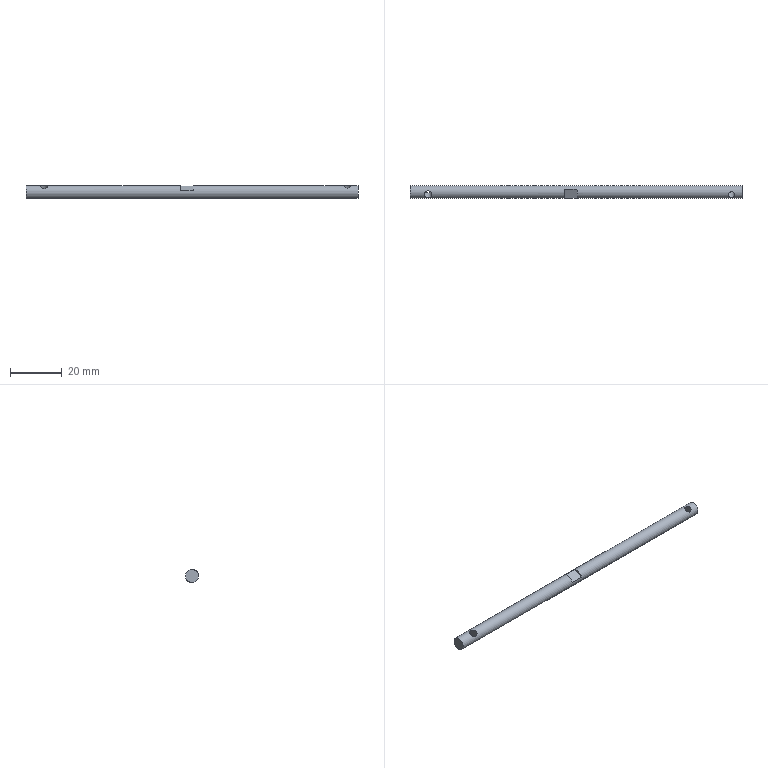Component | NX | 23B__27 | 1 solid | 8 faces | volume 2442 mm3 | plane 5 | cylinder 3 | commonest cylinder face diameters 5 x1 3 x1 2.5 x1